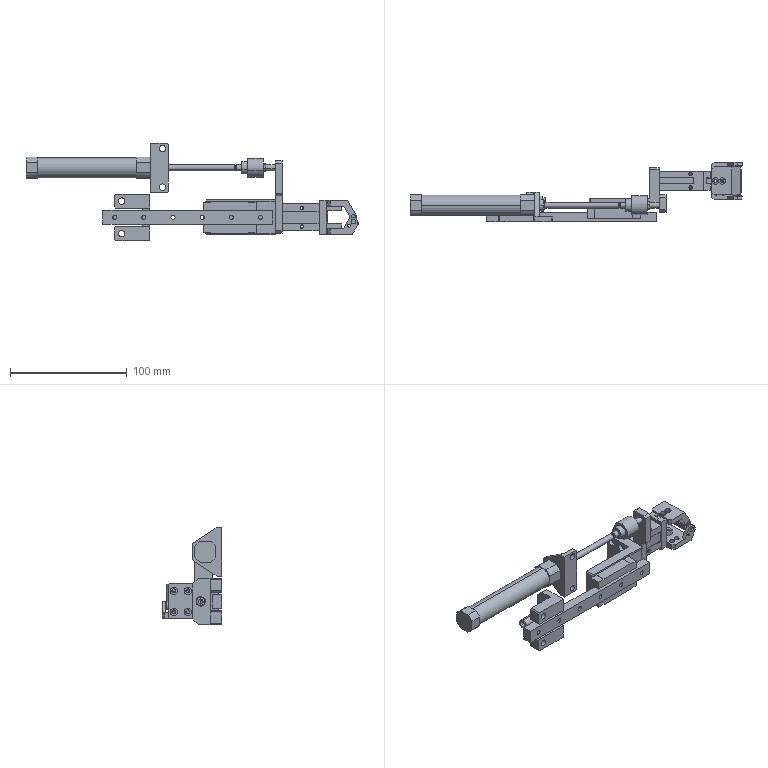Assembly | SolidWorks | mm | 18 component files | 19 solids | 629 faces | box 284.6 x 50.9 x 83.5 mm | volume 113198 mm3 | plane 271 | cylinder 235 | cone 123 | commonest cylinder face diameters 7 x31 2.46 x20 5.5 x16 3.4 x16 6.5 x16 5 x14 3.5 x12 6 x12
Bill of materials:
30604270309Roller | 1 | Teflon | Hollow cylindrical tube with a series of circumferential V-profile ridges along its middle length and plain cylindrical lands at both ends.
31298011300CylinderMountingPlate | 1 | Q235-A | L-shaped angle bracket with two plate legs at right angles, both drilled with several holes.
312981193FloatingJointConnection | 1 | Q235-A | Flat bar or link plate of constant thickness with a stepped, offset outline and three through holes.
312981493LimitBlock | 1 | Plain Carbon Steel | U- or C-shaped block made of two parallel arms joined by a back web. Each arm has a through hole, and the web has a larger hole on a perpendicular axis.
31298290203SupportFinger | 1 | Q235-A | Rectangular base plate with six through holes and two upright lugs at one end. The lugs have rounded tops and each carries a larger and a smaller hole.
31298300012MechanicalFinger | 1 | Q235-A | Bent, constant-section block: a flat top portion with two through holes, then an angled leg that ends in an open semicircular notch at its tip.
60100040019CylinderSupport | 1 | Q235-A | Angle bracket: a rectangular plate with two holes joined at right angles to a tapered, trapezoidal plate with one large hole.
60100060002HeadlessBufferScrewM8_40 | 1 | 45 | Solid cylindrical pin with chamfered ends and a short, smaller-diameter coaxial stub at one end.
CopyBody_A_CDJ2B16_60_B_0 | 1 |  | Elongated standoff-like part: a round central shaft between two polygonal (flat-sided) end sections, with a small cylindrical stub at one end that has an axial hole.
CopyRod_A_CDJ2B16_60_B_0 | 1 |  | Long, slender solid cylindrical rod with a narrow circumferential groove near one end and chamfered ends.
JA15_5_080 | 1 | 45 | Stepped coaxial turned part: a short pilot cylinder, a large cylindrical body, a small polygonal collar, then a chamfered cylindrical shaft.
MGN12H | 1 | Plain Carbon Steel | Elongated prismatic bar with a full-length rectangular channel on one face, giving a C-shaped cross-section. The middle portion is slightly taller than the end portions.
MGN12H145 | 1 | Plain Carbon Steel | Long, slender bar with a rectangular cross-section. A single row of six evenly spaced round holes runs along its length on one long face.
CopyBodyA_MHZ2-10D(11.2) | 1 |  | Rectangular block with a lengthwise slot or channel cut into its top, a thin lengthwise groove along one side face, and a wider stepped flange at one end. The flange has a rectangular notch. The block has round holes on its top and side faces.
OpticalAxis_4_32 | 1 | Q235-A | Plain solid round rod or pin: a straight cylinder with flat ends.
SiliconeStrip3x24 | 1 | Q235-A | Straight solid rod with a mostly round cross-section, plus a concave, curved cut running its full length along one side.
Mates:
1. concentric | MHZ2-10D-1/CopyCopyFinger2A_MHZ2-10D(11.2)-1 face at (192.17, 43.668, 45.929) dir (0, 0, -1) r 1.005 | 31298300012MechanicalFinger-1 face at (192.17, 43.668, 52.929) dir (0, 0, 1) r 1.45
2. parallel | MHZ2-10D-1/CopyCopyFinger2A_MHZ2-10D(11.2)-1 face at (200.87, 46.168, 47.929) dir (1, 0, 0) | 31298300012MechanicalFinger-1 face at (188.87, 31.668, 47.929) dir (-1, 0, 0)
3. concentric | MHZ2-10D-1/CopyBodyA_MHZ2-10D(11.2)-1 face at (147.655, 37.768, 47.329) dir (1, 0, 0) r 1.23 | 31298011300CylinderMountingPlate-2 face at (135.77, 37.768, 47.329) dir (1, 0, 0) r 3.25
4. concentric | MHZ2-10D-1/CopyBodyA_MHZ2-10D(11.2)-1 edge at (144.04, 49.768, 29.329) dir (-1, 0, 0) r 1.23 | 31298011300CylinderMountingPlate-2 face at (135.77, 49.768, 29.329) dir (1, 0, 0) r 3.25
5. coincident | MHZ2-10D-1/CopyBodyA_MHZ2-10D(11.2)-1 face at (143.77, 43.768, 38.329) dir (-1, 0, 0) | 31298011300CylinderMountingPlate-2 face at (143.77, 20.768, 53.329) dir (1, 0, 0)
6. coincident | 31298011300CylinderMountingPlate-2 face at (143.77, 20.768, 53.329) dir (1, 0, 0) | 312981193FloatingJointConnection-1 face at (143.77, 21.768, 56.829) dir (-1, 0, 0)
7. concentric | 31298011300CylinderMountingPlate-2 face at (94.77, 28.768, 48.329) dir (0, 1, 0) r 1.7 | MGN12H1R145Z0C-1/MGN12H-1 face at (94.77, 17.768, 48.329) dir (0, 1, 0) r 1.15
8. parallel | 31298011300CylinderMountingPlate-2 face at (83.77, 20.768, 23.329) dir (0, 0, -1) | MGN12H1R145Z0C-1/MGN12H-1 face at (82.07, 21.768, 24.829) dir (0, 0, -1)
9. concentric | 31298011300CylinderMountingPlate-2 face at (143.77, 26.768, 30.829) dir (1, 0, 0) r 1.65 | 312981193FloatingJointConnection-1 face at (149.77, 26.768, 30.829) dir (1, 0, 0) r 2.25
10. coincident | 312981493LimitBlock-1 face at (6.27, 8.768, 18.329) dir (0, -1, 0) | MGN12H1R145Z0C-1/MGN12H145-1 face at (141.27, 8.768, 44.329) dir (0, -1, 0)
11. parallel | 312981493LimitBlock-1 face at (6.27, 33.768, 18.329) dir (0, 0, -1) | MGN12H1R145Z0C-1/MGN12H145-1 face at (141.27, 16.768, 32.329) dir (0, 0, -1)
12. width | 312981493LimitBlock-1 face at (6.27, 33.768, 18.329) dir (0, 0, -1) | 312981493LimitBlock-1 face at (6.27, 33.768, 58.329) dir (0, 0, 1) | MGN12H1R145Z0C-1/MGN12H145-1 face at (141.27, 16.768, 32.329) dir (0, 0, -1) | MGN12H1R145Z0C-1/MGN12H145-1 face at (141.27, 16.768, 44.329) dir (0, 0, 1)
13. concentric | 312981493LimitBlock-1 face at (30.27, 26.768, 38.329) dir (-1, 0, 0) r 4 | 60100060002HeadlessBufferScrewM8_40-1 face at (4.492, 26.768, 38.329) dir (-1, 0, 0) r 4
14. distance | 60100060002HeadlessBufferScrewM8_40-1 face at (46.27, 26.768, 38.329) dir (1, 0, 0) | 312981493LimitBlock-1 face at (36.27, 33.768, 58.329) dir (1, 0, 0)
15. coincident | MGN12H1R145Z0C-1/MGN12H145-1 face at (141.27, 8.768, 44.329) dir (0, -1, 0) | 60100040019CylinderSupport-1 face at (41.27, 8.768, 101.829) dir (0, -1, 0)
16. distance | 60100040019CylinderSupport-1 face at (37.27, 8.768, 101.829) dir (-1, 0, 0) | MGN12H1R145Z0C-1/MGN12H145-1 face at (-3.73, 8.768, 44.329) dir (-1, 0, 0)
17. distance | 60100040019CylinderSupport-1 face at (41.27, 12.768, 59.829) dir (0, 0, -1) | MGN12H1R145Z0C-1/MGN12H145-1 face at (141.27, 16.768, 44.329) dir (0, 0, 1)
18. distance | 312981493LimitBlock-1 face at (6.27, 33.768, 58.329) dir (-1, 0, 0) | MGN12H1R145Z0C-1/MGN12H145-1 face at (-3.73, 8.768, 44.329) dir (-1, 0, 0)
19. parallel | 31298011300CylinderMountingPlate-2 face at (83.77, 20.768, 23.329) dir (0, 0, -1) | 312981193FloatingJointConnection-1 face at (149.77, 31.768, 24.829) dir (0, 0, -1)
20. coincident | 31298011300CylinderMountingPlate-2 face at (143.77, 21.768, 51.829) dir (0, -1, 0) | MGN12H1R145Z0C-1/MGN12H-1 face at (82.07, 21.768, 24.829) dir (0, 1, 0)
21. coincident | MHZ2-10D-1/CopyCopyFinger2A_MHZ2-10D(11.2)-1 face at (188.87, 46.168, 47.929) dir (0, 0, 1) | 31298300012MechanicalFinger-1 face at (202.697, 31.668, 47.929) dir (0, 0, -1)
22. concentric | 30604270309Roller-1 face at (210.87, 56.418, 34.729) dir (0, -1, 0) r 3.5 | OpticalAxis_4_32-1 face at (210.87, 27.668, 34.729) dir (0, 1, 0) r 2
23. width | OpticalAxis_4_32-1 face at (210.87, 59.668, 34.729) dir (0, 1, 0) | OpticalAxis_4_32-1 face at (210.87, 27.668, 34.729) dir (0, -1, 0) | 30604270309Roller-1 face at (210.87, 30.918, 34.729) dir (0, -1, 0) | 30604270309Roller-1 face at (210.87, 56.418, 34.729) dir (0, 1, 0)
24. coincident | MHZ2-10D-1/CopyCopyFinger1A_MHZ2-10D(11.2)-1 face at (200.87, 46.168, 28.729) dir (0, 0, -1) | 31298290203SupportFinger-1 face at (202.385, 59.668, 28.729) dir (0, 0, 1)
25. concentric | MHZ2-10D-1/CopyCopyFinger1A_MHZ2-10D(11.2)-1 face at (192.17, 43.668, 30.729) dir (0, 0, -1) r 1.005 | 31298290203SupportFinger-1 face at (192.17, 43.668, 23.729) dir (0, 0, -1) r 2.75
26. parallel | MHZ2-10D-1/CopyBodyA_MHZ2-10D(11.2)-1 face at (181.57, 43.768, 38.329) dir (-1, 0, 0) | 31298290203SupportFinger-1 face at (188.87, 59.668, 28.729) dir (-1, 0, 0)
27. concentric | OpticalAxis_4_32-1 face at (210.87, 27.668, 34.729) dir (0, 1, 0) r 2 | 31298290203SupportFinger-1 face at (210.87, 59.668, 34.729) dir (0, -1, 0) r 2
28. concentric | 31298300012MechanicalFinger-1 face at (210.87, 55.668, 38.929) dir (0, -1, 0) r 1.9 | SiliconeStrip3x24-1 face at (210.87, 31.668, 38.929) dir (0, 1, 0) r 1.9
29. coincident | 31298300012MechanicalFinger-1 face at (188.87, 31.668, 52.929) dir (0, -1, 0) | SiliconeStrip3x24-1 face at (210.87, 31.668, 38.929) dir (0, -1, 0)
30. concentric | 60100040019CylinderSupport-1 face at (37.27, 22.768, 80.829) dir (1, 0, 0) r 5.5 | A_CDJ2B16_60_B_0-1/CopyBody_A_CDJ2B16_60_B_0-1 face at (-69.48, 22.768, 80.829) dir (1, 0, 0) r 5
31. coincident | 60100040019CylinderSupport-1 face at (37.27, 8.768, 101.829) dir (-1, 0, 0) | A_CDJ2B16_60_B_0-1/CopyBody_A_CDJ2B16_60_B_0-1 face at (37.27, 22.768, 80.829) dir (1, 0, 0)
32. concentric | assembly face at (27.031, 22.768, 80.829) dir (1, 0, 0) r 2.5 | JA15_5_080-2 face at (115.27, 22.768, 80.829) dir (-1, 0, 0) r 8
33. distance | JA15_5_080-2 face at (115.27, 24.209, 75.694) dir (-1, 0, 0) | assembly face at (108.031, 22.768, 80.829) dir (1, 0, 0)
34. coincident | 312981193FloatingJointConnection-1 face at (149.77, 21.768, 56.829) dir (1, 0, 0) | JA15_5_080-2 face at (149.77, 22.768, 80.829) dir (1, 0, 0)
35. distance | A_CDJ2B16_60_B_0-1/CopyRod_A_CDJ2B16_60_B_0-1 face at (125.27, 22.768, 80.829) dir (1, 0, 0) | JA15_5_080-2 face at (115.27, 24.209, 75.694) dir (-1, 0, 0)
36. concentric | A_CDJ2B16_60_B_0-1/CopyRod_A_CDJ2B16_60_B_0-1 face at (44.27, 22.768, 80.829) dir (1, 0, 0) r 2.5 | JA15_5_080-2 face at (115.27, 22.768, 80.829) dir (-1, 0, 0) r 8
37. concentric | CopyBody_A_CDJ2B16_60_B_0-1 face at (0, 0, -114.75) dir (0, 0, 1) r 5 | CopyRod_A_CDJ2B16_60_B_0-1 face at (0, 0, -1) dir (0, 0, 1) r 2.5
38. distance | CopyRod_A_CDJ2B16_60_B_0-1 face at (0, 0, 80) dir (0, 0, 1) | CopyBody_A_CDJ2B16_60_B_0-1 face at (0, 0, -8) dir (0, 0, 1)
39. coincident | MGN12H145-1 face at (-2.255, -3.353, 6) dir (0, 1, 0) | MGN12H-1 face at (-81.133, -3.353, -6) dir (0, -1, 0)
40. coincident | MGN12H145-1 face at (-2.255, -3.353, 6) dir (0, 0, 1) | MGN12H-1 face at (-81.133, -3.353, 6) dir (0, 0, -1)
41. coincident | CopyCopyFinger1A_MHZ2-10D(11.2)-1 face at (-0.02537, 2.064, 0.1) dir (0, 1, 0) | CopyCopyFinger2A_MHZ2-10D(11.2)-1 face at (-0.02537, 2.064, 0.1) dir (0, 1, 0)
42. coincident | CopyCopyFinger1A_MHZ2-10D(11.2)-1 face at (0.07463, 2.064, 1.3) dir (0, 0, 1) | CopyCopyFinger2A_MHZ2-10D(11.2)-1 face at (-5.625, 2.064, 1.3) dir (0, 0, 1)
43. coincident | CopyBodyA_MHZ2-10D(11.2)-1 face at (31.475, -2.936, -3) dir (0, 0, 1) | CopyCopyFinger2A_MHZ2-10D(11.2)-1 face at (-0.1254, 2.064, -3) dir (0, 0, -1)
44. parallel | CopyCopyFinger1A_MHZ2-10D(11.2)-1 face at (0.07463, 2.064, -3) dir (-1, 0, 0) | CopyCopyFinger2A_MHZ2-10D(11.2)-1 face at (-0.1254, 2.064, 1.3) dir (1, 0, 0)
45. coincident | CopyBodyA_MHZ2-10D(11.2)-1 face at (31.475, -2.936, 1.2) dir (0, 1, 0) | CopyCopyFinger1A_MHZ2-10D(11.2)-1 face at (-0.02537, -2.936, 0.1) dir (0, -1, 0)
46. distance | CopyCopyFinger1A_MHZ2-10D(11.2)-1 face at (12.475, 2.064, 1.3) dir (1, 0, 0) | CopyBodyA_MHZ2-10D(11.2)-1 face at (14.475, -8.536, 0) dir (1, 0, 0)
47. distance | CopyCopyFinger2A_MHZ2-10D(11.2)-1 face at (-12.525, 2.064, -3) dir (-1, 0, 0) | CopyBodyA_MHZ2-10D(11.2)-1 face at (-14.525, 7.864, 0) dir (-1, 0, 0)